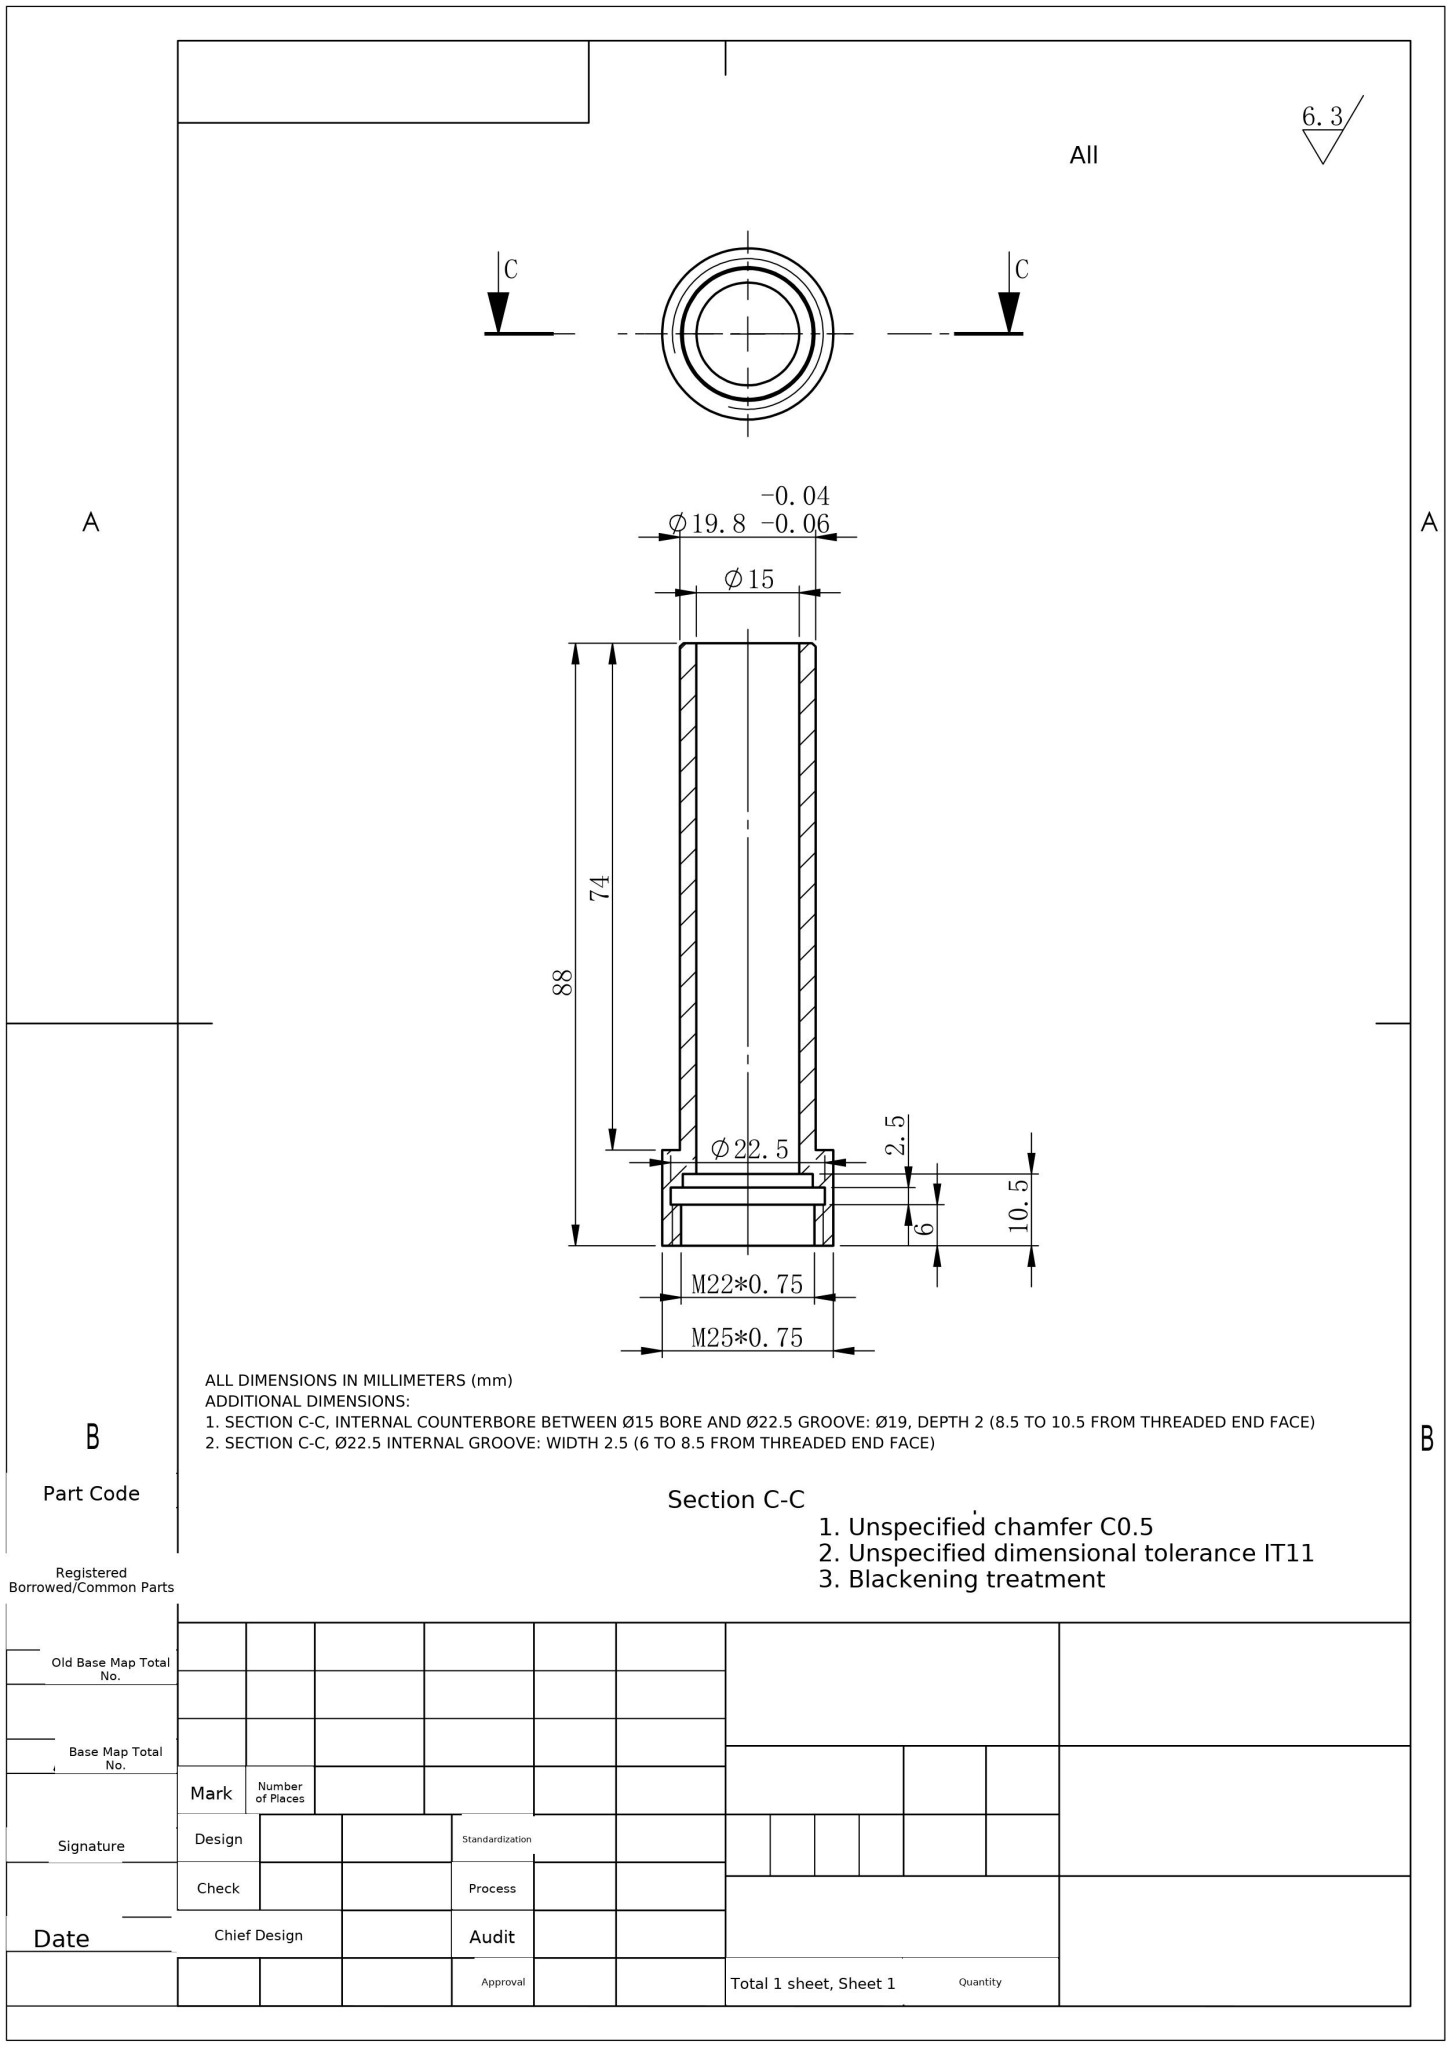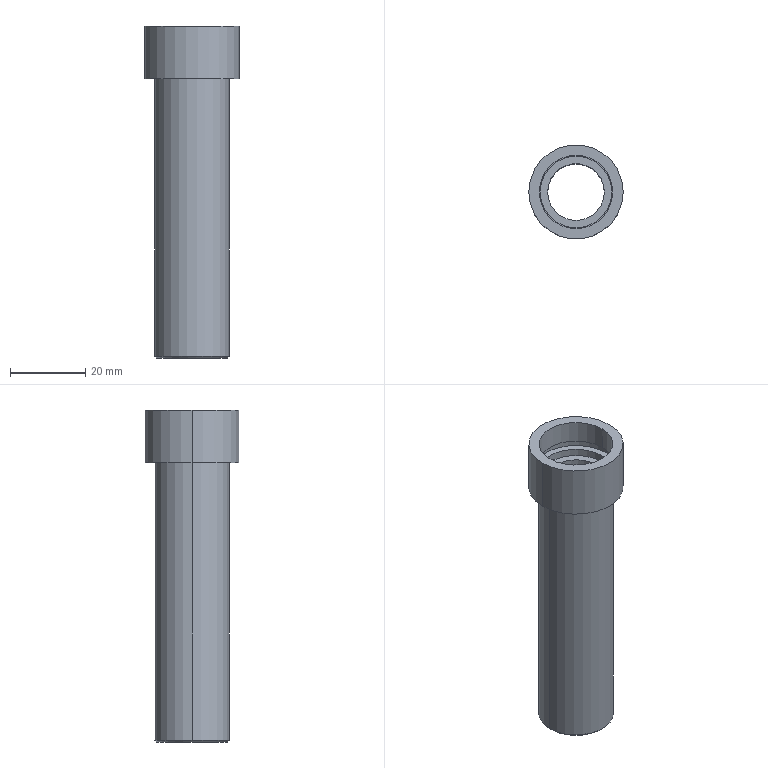Part | NX | mm | 1 solid | 20 faces | box 25 x 25 x 88 mm | volume 12601 mm3 | cylinder 12 | plane 6 | cone 2 | commonest cylinder face diameters 19 x2 25 x2 15 x2 19.8 x2 19.5 x2 22.5 x2
STEP:
#1=COLOUR_RGB('',0.5294,0.549,0.549);
#2=FILL_AREA_STYLE_COLOUR('',#1);
#3=FILL_AREA_STYLE('',(#2));
#4=SURFACE_STYLE_FILL_AREA(#3);
#5=SURFACE_SIDE_STYLE('',(#4));
#6=SURFACE_STYLE_USAGE(.BOTH.,#5);
#7=PRESENTATION_STYLE_ASSIGNMENT((#6));
#8=CARTESIAN_POINT('',(-9.4,0.,0.));
#9=VERTEX_POINT('',#8);
#10=CARTESIAN_POINT('',(9.4,0.,0.));
#11=VERTEX_POINT('',#10);
#12=CARTESIAN_POINT('',(0.,0.,0.));
#13=DIRECTION('',(0.,0.,-1.));
#14=DIRECTION('',(1.,0.,0.));
#15=AXIS2_PLACEMENT_3D('',#12,#13,#14);
#16=CIRCLE('',#15,9.4);
#17=EDGE_CURVE('',#9,#11,#16,.T.);
#18=ORIENTED_EDGE('',*,*,#17,.F.);
#19=CARTESIAN_POINT('',(-9.9,0.,0.5));
#20=VERTEX_POINT('',#19);
#21=CARTESIAN_POINT('',(-9.9,0.,0.5));
#22=DIRECTION('',(-0.7071,0.,0.7071));
#23=VECTOR('',#22,1000.);
#24=LINE('',#21,#23);
#25=EDGE_CURVE('',#9,#20,#24,.T.);
#26=ORIENTED_EDGE('',*,*,#25,.T.);
#27=CARTESIAN_POINT('',(9.9,0.,0.5));
#28=VERTEX_POINT('',#27);
#29=CARTESIAN_POINT('',(0.,0.,0.5));
#30=DIRECTION('',(0.,0.,1.));
#31=DIRECTION('',(1.,0.,0.));
#32=AXIS2_PLACEMENT_3D('',#29,#30,#31);
#33=CIRCLE('',#32,9.9);
#34=EDGE_CURVE('',#28,#20,#33,.T.);
#35=ORIENTED_EDGE('',*,*,#34,.F.);
#36=CARTESIAN_POINT('',(9.9,0.,0.5));
#37=DIRECTION('',(0.7071,0.,0.7071));
#38=VECTOR('',#37,1000.);
#39=LINE('',#36,#38);
#40=EDGE_CURVE('',#11,#28,#39,.T.);
#41=ORIENTED_EDGE('',*,*,#40,.F.);
#42=EDGE_LOOP('',(#18,#26,#35,#41));
#43=FACE_OUTER_BOUND('',#42,.T.);
#44=CARTESIAN_POINT('',(0.,0.,0.5));
#45=DIRECTION('',(0.,0.,1.));
#46=DIRECTION('',(1.,0.,0.));
#47=AXIS2_PLACEMENT_3D('',#44,#45,#46);
#48=CONICAL_SURFACE('',#47,9.9,0.7854);
#49=ADVANCED_FACE('',(#43),#48,.T.);
#50=CARTESIAN_POINT('',(-9.5,0.,77.5));
#51=VERTEX_POINT('',#50);
#52=CARTESIAN_POINT('',(9.5,0.,77.5));
#53=VERTEX_POINT('',#52);
#54=CARTESIAN_POINT('',(0.,0.,77.5));
#55=DIRECTION('',(0.,0.,1.));
#56=DIRECTION('',(1.,0.,0.));
#57=AXIS2_PLACEMENT_3D('',#54,#55,#56);
#58=CIRCLE('',#57,9.5);
#59=EDGE_CURVE('',#51,#53,#58,.T.);
#60=ORIENTED_EDGE('',*,*,#59,.F.);
#61=CARTESIAN_POINT('',(-9.5,0.,79.5));
#62=VERTEX_POINT('',#61);
#63=CARTESIAN_POINT('',(-9.5,0.,77.5));
#64=DIRECTION('',(0.,0.,1.));
#65=VECTOR('',#64,1000.);
#66=LINE('',#63,#65);
#67=EDGE_CURVE('',#51,#62,#66,.T.);
#68=ORIENTED_EDGE('',*,*,#67,.T.);
#69=CARTESIAN_POINT('',(9.5,0.,79.5));
#70=VERTEX_POINT('',#69);
#71=CARTESIAN_POINT('',(0.,0.,79.5));
#72=DIRECTION('',(0.,0.,1.));
#73=DIRECTION('',(1.,0.,0.));
#74=AXIS2_PLACEMENT_3D('',#71,#72,#73);
#75=CIRCLE('',#74,9.5);
#76=EDGE_CURVE('',#62,#70,#75,.T.);
#77=ORIENTED_EDGE('',*,*,#76,.T.);
#78=CARTESIAN_POINT('',(9.5,0.,77.5));
#79=DIRECTION('',(0.,0.,1.));
#80=VECTOR('',#79,1000.);
#81=LINE('',#78,#80);
#82=EDGE_CURVE('',#53,#70,#81,.T.);
#83=ORIENTED_EDGE('',*,*,#82,.F.);
#84=EDGE_LOOP('',(#60,#68,#77,#83));
#85=FACE_OUTER_BOUND('',#84,.T.);
#86=CARTESIAN_POINT('',(0.,0.,77.5));
#87=DIRECTION('',(0.,0.,1.));
#88=DIRECTION('',(1.,0.,0.));
#89=AXIS2_PLACEMENT_3D('',#86,#87,#88);
#90=CYLINDRICAL_SURFACE('',#89,9.5);
#91=ADVANCED_FACE('',(#85),#90,.F.);
#92=CARTESIAN_POINT('',(12.5,0.,88.));
#93=VERTEX_POINT('',#92);
#94=CARTESIAN_POINT('',(-12.5,0.,88.));
#95=VERTEX_POINT('',#94);
#96=CARTESIAN_POINT('',(0.,0.,88.));
#97=DIRECTION('',(0.,0.,1.));
#98=DIRECTION('',(1.,0.,0.));
#99=AXIS2_PLACEMENT_3D('',#96,#97,#98);
#100=CIRCLE('',#99,12.5);
#101=EDGE_CURVE('',#93,#95,#100,.T.);
#102=ORIENTED_EDGE('',*,*,#101,.F.);
#103=CARTESIAN_POINT('',(12.5,0.,74.));
#104=VERTEX_POINT('',#103);
#105=CARTESIAN_POINT('',(12.5,0.,88.));
#106=DIRECTION('',(0.,0.,-1.));
#107=VECTOR('',#106,1000.);
#108=LINE('',#105,#107);
#109=EDGE_CURVE('',#93,#104,#108,.T.);
#110=ORIENTED_EDGE('',*,*,#109,.T.);
#111=CARTESIAN_POINT('',(-12.5,0.,74.));
#112=VERTEX_POINT('',#111);
#113=CARTESIAN_POINT('',(0.,0.,74.));
#114=DIRECTION('',(0.,0.,1.));
#115=DIRECTION('',(1.,0.,0.));
#116=AXIS2_PLACEMENT_3D('',#113,#114,#115);
#117=CIRCLE('',#116,12.5);
#118=EDGE_CURVE('',#104,#112,#117,.T.);
#119=ORIENTED_EDGE('',*,*,#118,.T.);
#120=CARTESIAN_POINT('',(-12.5,0.,88.));
#121=DIRECTION('',(0.,0.,-1.));
#122=VECTOR('',#121,1000.);
#123=LINE('',#120,#122);
#124=EDGE_CURVE('',#95,#112,#123,.T.);
#125=ORIENTED_EDGE('',*,*,#124,.F.);
#126=EDGE_LOOP('',(#102,#110,#119,#125));
#127=FACE_OUTER_BOUND('',#126,.T.);
#128=CARTESIAN_POINT('',(0.,0.,88.));
#129=DIRECTION('',(0.,0.,-1.));
#130=DIRECTION('',(-1.,0.,0.));
#131=AXIS2_PLACEMENT_3D('',#128,#129,#130);
#132=CYLINDRICAL_SURFACE('',#131,12.5);
#133=ADVANCED_FACE('',(#127),#132,.T.);
#134=CARTESIAN_POINT('',(-7.5,0.,77.5));
#135=VERTEX_POINT('',#134);
#136=CARTESIAN_POINT('',(7.5,0.,77.5));
#137=VERTEX_POINT('',#136);
#138=CARTESIAN_POINT('',(0.,0.,77.5));
#139=DIRECTION('',(0.,0.,1.));
#140=DIRECTION('',(1.,0.,0.));
#141=AXIS2_PLACEMENT_3D('',#138,#139,#140);
#142=CIRCLE('',#141,7.5);
#143=EDGE_CURVE('',#135,#137,#142,.T.);
#144=ORIENTED_EDGE('',*,*,#143,.T.);
#145=CARTESIAN_POINT('',(7.5,0.,0.));
#146=VERTEX_POINT('',#145);
#147=CARTESIAN_POINT('',(7.5,0.,74.));
#148=DIRECTION('',(0.,0.,-1.));
#149=VECTOR('',#148,1000.);
#150=LINE('',#147,#149);
#151=EDGE_CURVE('',#137,#146,#150,.T.);
#152=ORIENTED_EDGE('',*,*,#151,.T.);
#153=CARTESIAN_POINT('',(-7.5,0.,0.));
#154=VERTEX_POINT('',#153);
#155=CARTESIAN_POINT('',(0.,0.,0.));
#156=DIRECTION('',(0.,0.,1.));
#157=DIRECTION('',(1.,0.,0.));
#158=AXIS2_PLACEMENT_3D('',#155,#156,#157);
#159=CIRCLE('',#158,7.5);
#160=EDGE_CURVE('',#154,#146,#159,.T.);
#161=ORIENTED_EDGE('',*,*,#160,.F.);
#162=CARTESIAN_POINT('',(-7.5,0.,74.));
#163=DIRECTION('',(0.,0.,-1.));
#164=VECTOR('',#163,1000.);
#165=LINE('',#162,#164);
#166=EDGE_CURVE('',#135,#154,#165,.T.);
#167=ORIENTED_EDGE('',*,*,#166,.F.);
#168=EDGE_LOOP('',(#144,#152,#161,#167));
#169=FACE_OUTER_BOUND('',#168,.T.);
#170=CARTESIAN_POINT('',(0.,0.,74.));
#171=DIRECTION('',(0.,0.,-1.));
#172=DIRECTION('',(-1.,0.,0.));
#173=AXIS2_PLACEMENT_3D('',#170,#171,#172);
#174=CYLINDRICAL_SURFACE('',#173,7.5);
#175=ADVANCED_FACE('',(#169),#174,.F.);
#176=CARTESIAN_POINT('',(9.9,0.,74.));
#177=VERTEX_POINT('',#176);
#178=CARTESIAN_POINT('',(-9.9,0.,74.));
#179=VERTEX_POINT('',#178);
#180=CARTESIAN_POINT('',(0.,0.,74.));
#181=DIRECTION('',(0.,0.,1.));
#182=DIRECTION('',(1.,0.,0.));
#183=AXIS2_PLACEMENT_3D('',#180,#181,#182);
#184=CIRCLE('',#183,9.9);
#185=EDGE_CURVE('',#177,#179,#184,.T.);
#186=ORIENTED_EDGE('',*,*,#185,.F.);
#187=CARTESIAN_POINT('',(9.9,0.,74.));
#188=DIRECTION('',(0.,0.,-1.));
#189=VECTOR('',#188,1000.);
#190=LINE('',#187,#189);
#191=EDGE_CURVE('',#177,#28,#190,.T.);
#192=ORIENTED_EDGE('',*,*,#191,.T.);
#193=ORIENTED_EDGE('',*,*,#34,.T.);
#194=CARTESIAN_POINT('',(-9.9,0.,74.));
#195=DIRECTION('',(0.,0.,-1.));
#196=VECTOR('',#195,1000.);
#197=LINE('',#194,#196);
#198=EDGE_CURVE('',#179,#20,#197,.T.);
#199=ORIENTED_EDGE('',*,*,#198,.F.);
#200=EDGE_LOOP('',(#186,#192,#193,#199));
#201=FACE_OUTER_BOUND('',#200,.T.);
#202=CARTESIAN_POINT('',(0.,0.,74.));
#203=DIRECTION('',(0.,0.,-1.));
#204=DIRECTION('',(-1.,0.,0.));
#205=AXIS2_PLACEMENT_3D('',#202,#203,#204);
#206=CYLINDRICAL_SURFACE('',#205,9.9);
#207=ADVANCED_FACE('',(#201),#206,.T.);
#208=CARTESIAN_POINT('',(-9.75,0.,82.));
#209=VERTEX_POINT('',#208);
#210=CARTESIAN_POINT('',(9.75,0.,82.));
#211=VERTEX_POINT('',#210);
#212=CARTESIAN_POINT('',(0.,0.,82.));
#213=DIRECTION('',(0.,0.,1.));
#214=DIRECTION('',(1.,0.,0.));
#215=AXIS2_PLACEMENT_3D('',#212,#213,#214);
#216=CIRCLE('',#215,9.75);
#217=EDGE_CURVE('',#209,#211,#216,.T.);
#218=ORIENTED_EDGE('',*,*,#217,.F.);
#219=CARTESIAN_POINT('',(-9.75,0.,88.));
#220=VERTEX_POINT('',#219);
#221=CARTESIAN_POINT('',(-9.75,0.,88.));
#222=DIRECTION('',(0.,0.,1.));
#223=VECTOR('',#222,1000.);
#224=LINE('',#221,#223);
#225=EDGE_CURVE('',#209,#220,#224,.T.);
#226=ORIENTED_EDGE('',*,*,#225,.T.);
#227=CARTESIAN_POINT('',(9.75,0.,88.));
#228=VERTEX_POINT('',#227);
#229=CARTESIAN_POINT('',(0.,0.,88.));
#230=DIRECTION('',(0.,0.,1.));
#231=DIRECTION('',(1.,0.,0.));
#232=AXIS2_PLACEMENT_3D('',#229,#230,#231);
#233=CIRCLE('',#232,9.75);
#234=EDGE_CURVE('',#220,#228,#233,.T.);
#235=ORIENTED_EDGE('',*,*,#234,.T.);
#236=CARTESIAN_POINT('',(9.75,0.,88.));
#237=DIRECTION('',(0.,0.,1.));
#238=VECTOR('',#237,1000.);
#239=LINE('',#236,#238);
#240=EDGE_CURVE('',#211,#228,#239,.T.);
#241=ORIENTED_EDGE('',*,*,#240,.F.);
#242=EDGE_LOOP('',(#218,#226,#235,#241));
#243=FACE_OUTER_BOUND('',#242,.T.);
#244=CARTESIAN_POINT('',(0.,0.,88.));
#245=DIRECTION('',(0.,0.,1.));
#246=DIRECTION('',(1.,0.,0.));
#247=AXIS2_PLACEMENT_3D('',#244,#245,#246);
#248=CYLINDRICAL_SURFACE('',#247,9.75);
#249=ADVANCED_FACE('',(#243),#248,.F.);
#250=CARTESIAN_POINT('',(-11.25,0.,79.5));
#251=VERTEX_POINT('',#250);
#252=CARTESIAN_POINT('',(11.25,0.,79.5));
#253=VERTEX_POINT('',#252);
#254=CARTESIAN_POINT('',(0.,0.,79.5));
#255=DIRECTION('',(0.,0.,1.));
#256=DIRECTION('',(1.,0.,0.));
#257=AXIS2_PLACEMENT_3D('',#254,#255,#256);
#258=CIRCLE('',#257,11.25);
#259=EDGE_CURVE('',#251,#253,#258,.T.);
#260=ORIENTED_EDGE('',*,*,#259,.F.);
#261=CARTESIAN_POINT('',(-11.25,0.,82.));
#262=VERTEX_POINT('',#261);
#263=CARTESIAN_POINT('',(-11.25,0.,79.5));
#264=DIRECTION('',(0.,0.,1.));
#265=VECTOR('',#264,1000.);
#266=LINE('',#263,#265);
#267=EDGE_CURVE('',#251,#262,#266,.T.);
#268=ORIENTED_EDGE('',*,*,#267,.T.);
#269=CARTESIAN_POINT('',(11.25,0.,82.));
#270=VERTEX_POINT('',#269);
#271=CARTESIAN_POINT('',(0.,0.,82.));
#272=DIRECTION('',(0.,0.,1.));
#273=DIRECTION('',(1.,0.,0.));
#274=AXIS2_PLACEMENT_3D('',#271,#272,#273);
#275=CIRCLE('',#274,11.25);
#276=EDGE_CURVE('',#262,#270,#275,.T.);
#277=ORIENTED_EDGE('',*,*,#276,.T.);
#278=CARTESIAN_POINT('',(11.25,0.,79.5));
#279=DIRECTION('',(0.,0.,1.));
#280=VECTOR('',#279,1000.);
#281=LINE('',#278,#280);
#282=EDGE_CURVE('',#253,#270,#281,.T.);
#283=ORIENTED_EDGE('',*,*,#282,.F.);
#284=EDGE_LOOP('',(#260,#268,#277,#283));
#285=FACE_OUTER_BOUND('',#284,.T.);
#286=CARTESIAN_POINT('',(0.,0.,79.5));
#287=DIRECTION('',(0.,0.,1.));
#288=DIRECTION('',(1.,0.,0.));
#289=AXIS2_PLACEMENT_3D('',#286,#287,#288);
#290=CYLINDRICAL_SURFACE('',#289,11.25);
#291=ADVANCED_FACE('',(#285),#290,.F.);
#292=ORIENTED_EDGE('',*,*,#267,.F.);
#293=CARTESIAN_POINT('',(0.,0.,79.5));
#294=DIRECTION('',(0.,0.,1.));
#295=DIRECTION('',(1.,0.,0.));
#296=AXIS2_PLACEMENT_3D('',#293,#294,#295);
#297=CIRCLE('',#296,11.25);
#298=EDGE_CURVE('',#253,#251,#297,.T.);
#299=ORIENTED_EDGE('',*,*,#298,.F.);
#300=ORIENTED_EDGE('',*,*,#282,.T.);
#301=CARTESIAN_POINT('',(0.,0.,82.));
#302=DIRECTION('',(0.,0.,1.));
#303=DIRECTION('',(1.,0.,0.));
#304=AXIS2_PLACEMENT_3D('',#301,#302,#303);
#305=CIRCLE('',#304,11.25);
#306=EDGE_CURVE('',#270,#262,#305,.T.);
#307=ORIENTED_EDGE('',*,*,#306,.T.);
#308=EDGE_LOOP('',(#292,#299,#300,#307));
#309=FACE_OUTER_BOUND('',#308,.T.);
#310=CARTESIAN_POINT('',(0.,0.,79.5));
#311=DIRECTION('',(0.,0.,1.));
#312=DIRECTION('',(1.,0.,0.));
#313=AXIS2_PLACEMENT_3D('',#310,#311,#312);
#314=CYLINDRICAL_SURFACE('',#313,11.25);
#315=ADVANCED_FACE('',(#309),#314,.F.);
#316=CARTESIAN_POINT('',(0.,0.,79.5));
#317=DIRECTION('',(0.,0.,1.));
#318=DIRECTION('',(1.,0.,0.));
#319=AXIS2_PLACEMENT_3D('',#316,#317,#318);
#320=CIRCLE('',#319,9.5);
#321=EDGE_CURVE('',#70,#62,#320,.T.);
#322=ORIENTED_EDGE('',*,*,#321,.F.);
#323=ORIENTED_EDGE('',*,*,#76,.F.);
#324=EDGE_LOOP('',(#322,#323));
#325=FACE_BOUND('',#324,.T.);
#326=ORIENTED_EDGE('',*,*,#298,.T.);
#327=ORIENTED_EDGE('',*,*,#259,.T.);
#328=EDGE_LOOP('',(#326,#327));
#329=FACE_OUTER_BOUND('',#328,.T.);
#330=CARTESIAN_POINT('',(0.,0.,79.5));
#331=DIRECTION('',(0.,0.,1.));
#332=DIRECTION('',(1.,0.,0.));
#333=AXIS2_PLACEMENT_3D('',#330,#331,#332);
#334=PLANE('',#333);
#335=ADVANCED_FACE('',(#325,#329),#334,.T.);
#336=CARTESIAN_POINT('',(0.,0.,82.));
#337=DIRECTION('',(0.,0.,1.));
#338=DIRECTION('',(1.,0.,0.));
#339=AXIS2_PLACEMENT_3D('',#336,#337,#338);
#340=CIRCLE('',#339,9.75);
#341=EDGE_CURVE('',#211,#209,#340,.T.);
#342=ORIENTED_EDGE('',*,*,#341,.T.);
#343=ORIENTED_EDGE('',*,*,#217,.T.);
#344=EDGE_LOOP('',(#342,#343));
#345=FACE_BOUND('',#344,.T.);
#346=ORIENTED_EDGE('',*,*,#306,.F.);
#347=ORIENTED_EDGE('',*,*,#276,.F.);
#348=EDGE_LOOP('',(#346,#347));
#349=FACE_OUTER_BOUND('',#348,.T.);
#350=CARTESIAN_POINT('',(0.,0.,82.));
#351=DIRECTION('',(0.,0.,1.));
#352=DIRECTION('',(1.,0.,0.));
#353=AXIS2_PLACEMENT_3D('',#350,#351,#352);
#354=PLANE('',#353);
#355=ADVANCED_FACE('',(#345,#349),#354,.F.);
#356=ORIENTED_EDGE('',*,*,#225,.F.);
#357=ORIENTED_EDGE('',*,*,#341,.F.);
#358=ORIENTED_EDGE('',*,*,#240,.T.);
#359=CARTESIAN_POINT('',(0.,0.,88.));
#360=DIRECTION('',(0.,0.,1.));
#361=DIRECTION('',(1.,0.,0.));
#362=AXIS2_PLACEMENT_3D('',#359,#360,#361);
#363=CIRCLE('',#362,9.75);
#364=EDGE_CURVE('',#228,#220,#363,.T.);
#365=ORIENTED_EDGE('',*,*,#364,.T.);
#366=EDGE_LOOP('',(#356,#357,#358,#365));
#367=FACE_OUTER_BOUND('',#366,.T.);
#368=CARTESIAN_POINT('',(0.,0.,88.));
#369=DIRECTION('',(0.,0.,1.));
#370=DIRECTION('',(1.,0.,0.));
#371=AXIS2_PLACEMENT_3D('',#368,#369,#370);
#372=CYLINDRICAL_SURFACE('',#371,9.75);
#373=ADVANCED_FACE('',(#367),#372,.F.);
#374=CARTESIAN_POINT('',(0.,0.,0.));
#375=DIRECTION('',(0.,0.,-1.));
#376=DIRECTION('',(1.,0.,0.));
#377=AXIS2_PLACEMENT_3D('',#374,#375,#376);
#378=CIRCLE('',#377,9.4);
#379=EDGE_CURVE('',#11,#9,#378,.T.);
#380=ORIENTED_EDGE('',*,*,#379,.T.);
#381=ORIENTED_EDGE('',*,*,#17,.T.);
#382=EDGE_LOOP('',(#380,#381));
#383=FACE_OUTER_BOUND('',#382,.T.);
#384=ORIENTED_EDGE('',*,*,#160,.T.);
#385=CARTESIAN_POINT('',(0.,0.,0.));
#386=DIRECTION('',(0.,0.,1.));
#387=DIRECTION('',(1.,0.,0.));
#388=AXIS2_PLACEMENT_3D('',#385,#386,#387);
#389=CIRCLE('',#388,7.5);
#390=EDGE_CURVE('',#146,#154,#389,.T.);
#391=ORIENTED_EDGE('',*,*,#390,.T.);
#392=EDGE_LOOP('',(#384,#391));
#393=FACE_BOUND('',#392,.T.);
#394=CARTESIAN_POINT('',(0.,0.,0.));
#395=DIRECTION('',(0.,0.,1.));
#396=DIRECTION('',(1.,0.,0.));
#397=AXIS2_PLACEMENT_3D('',#394,#395,#396);
#398=PLANE('',#397);
#399=ADVANCED_FACE('',(#383,#393),#398,.F.);
#400=ORIENTED_EDGE('',*,*,#191,.F.);
#401=CARTESIAN_POINT('',(0.,0.,74.));
#402=DIRECTION('',(0.,0.,1.));
#403=DIRECTION('',(1.,0.,0.));
#404=AXIS2_PLACEMENT_3D('',#401,#402,#403);
#405=CIRCLE('',#404,9.9);
#406=EDGE_CURVE('',#179,#177,#405,.T.);
#407=ORIENTED_EDGE('',*,*,#406,.F.);
#408=ORIENTED_EDGE('',*,*,#198,.T.);
#409=CARTESIAN_POINT('',(0.,0.,0.5));
#410=DIRECTION('',(0.,0.,1.));
#411=DIRECTION('',(1.,0.,0.));
#412=AXIS2_PLACEMENT_3D('',#409,#410,#411);
#413=CIRCLE('',#412,9.9);
#414=EDGE_CURVE('',#20,#28,#413,.T.);
#415=ORIENTED_EDGE('',*,*,#414,.T.);
#416=EDGE_LOOP('',(#400,#407,#408,#415));
#417=FACE_OUTER_BOUND('',#416,.T.);
#418=CARTESIAN_POINT('',(0.,0.,74.));
#419=DIRECTION('',(0.,0.,-1.));
#420=DIRECTION('',(-1.,0.,0.));
#421=AXIS2_PLACEMENT_3D('',#418,#419,#420);
#422=CYLINDRICAL_SURFACE('',#421,9.9);
#423=ADVANCED_FACE('',(#417),#422,.T.);
#424=ORIENTED_EDGE('',*,*,#151,.F.);
#425=CARTESIAN_POINT('',(0.,0.,77.5));
#426=DIRECTION('',(0.,0.,1.));
#427=DIRECTION('',(1.,0.,0.));
#428=AXIS2_PLACEMENT_3D('',#425,#426,#427);
#429=CIRCLE('',#428,7.5);
#430=EDGE_CURVE('',#137,#135,#429,.T.);
#431=ORIENTED_EDGE('',*,*,#430,.T.);
#432=ORIENTED_EDGE('',*,*,#166,.T.);
#433=ORIENTED_EDGE('',*,*,#390,.F.);
#434=EDGE_LOOP('',(#424,#431,#432,#433));
#435=FACE_OUTER_BOUND('',#434,.T.);
#436=CARTESIAN_POINT('',(0.,0.,74.));
#437=DIRECTION('',(0.,0.,-1.));
#438=DIRECTION('',(-1.,0.,0.));
#439=AXIS2_PLACEMENT_3D('',#436,#437,#438);
#440=CYLINDRICAL_SURFACE('',#439,7.5);
#441=ADVANCED_FACE('',(#435),#440,.F.);
#442=CARTESIAN_POINT('',(0.,0.,74.));
#443=DIRECTION('',(0.,0.,1.));
#444=DIRECTION('',(1.,0.,0.));
#445=AXIS2_PLACEMENT_3D('',#442,#443,#444);
#446=CIRCLE('',#445,12.5);
#447=EDGE_CURVE('',#112,#104,#446,.T.);
#448=ORIENTED_EDGE('',*,*,#447,.F.);
#449=ORIENTED_EDGE('',*,*,#118,.F.);
#450=EDGE_LOOP('',(#448,#449));
#451=FACE_OUTER_BOUND('',#450,.T.);
#452=ORIENTED_EDGE('',*,*,#406,.T.);
#453=ORIENTED_EDGE('',*,*,#185,.T.);
#454=EDGE_LOOP('',(#452,#453));
#455=FACE_BOUND('',#454,.T.);
#456=CARTESIAN_POINT('',(0.,0.,74.));
#457=DIRECTION('',(0.,0.,1.));
#458=DIRECTION('',(1.,0.,0.));
#459=AXIS2_PLACEMENT_3D('',#456,#457,#458);
#460=PLANE('',#459);
#461=ADVANCED_FACE('',(#451,#455),#460,.F.);
#462=ORIENTED_EDGE('',*,*,#109,.F.);
#463=CARTESIAN_POINT('',(0.,0.,88.));
#464=DIRECTION('',(0.,0.,1.));
#465=DIRECTION('',(1.,0.,0.));
#466=AXIS2_PLACEMENT_3D('',#463,#464,#465);
#467=CIRCLE('',#466,12.5);
#468=EDGE_CURVE('',#95,#93,#467,.T.);
#469=ORIENTED_EDGE('',*,*,#468,.F.);
#470=ORIENTED_EDGE('',*,*,#124,.T.);
#471=ORIENTED_EDGE('',*,*,#447,.T.);
#472=EDGE_LOOP('',(#462,#469,#470,#471));
#473=FACE_OUTER_BOUND('',#472,.T.);
#474=CARTESIAN_POINT('',(0.,0.,88.));
#475=DIRECTION('',(0.,0.,-1.));
#476=DIRECTION('',(-1.,0.,0.));
#477=AXIS2_PLACEMENT_3D('',#474,#475,#476);
#478=CYLINDRICAL_SURFACE('',#477,12.5);
#479=ADVANCED_FACE('',(#473),#478,.T.);
#480=ORIENTED_EDGE('',*,*,#364,.F.);
#481=ORIENTED_EDGE('',*,*,#234,.F.);
#482=EDGE_LOOP('',(#480,#481));
#483=FACE_BOUND('',#482,.T.);
#484=ORIENTED_EDGE('',*,*,#468,.T.);
#485=ORIENTED_EDGE('',*,*,#101,.T.);
#486=EDGE_LOOP('',(#484,#485));
#487=FACE_OUTER_BOUND('',#486,.T.);
#488=CARTESIAN_POINT('',(0.,0.,88.));
#489=DIRECTION('',(0.,0.,1.));
#490=DIRECTION('',(1.,0.,0.));
#491=AXIS2_PLACEMENT_3D('',#488,#489,#490);
#492=PLANE('',#491);
#493=ADVANCED_FACE('',(#483,#487),#492,.T.);
#494=ORIENTED_EDGE('',*,*,#67,.F.);
#495=CARTESIAN_POINT('',(0.,0.,77.5));
#496=DIRECTION('',(0.,0.,1.));
#497=DIRECTION('',(1.,0.,0.));
#498=AXIS2_PLACEMENT_3D('',#495,#496,#497);
#499=CIRCLE('',#498,9.5);
#500=EDGE_CURVE('',#53,#51,#499,.T.);
#501=ORIENTED_EDGE('',*,*,#500,.F.);
#502=ORIENTED_EDGE('',*,*,#82,.T.);
#503=ORIENTED_EDGE('',*,*,#321,.T.);
#504=EDGE_LOOP('',(#494,#501,#502,#503));
#505=FACE_OUTER_BOUND('',#504,.T.);
#506=CARTESIAN_POINT('',(0.,0.,77.5));
#507=DIRECTION('',(0.,0.,1.));
#508=DIRECTION('',(1.,0.,0.));
#509=AXIS2_PLACEMENT_3D('',#506,#507,#508);
#510=CYLINDRICAL_SURFACE('',#509,9.5);
#511=ADVANCED_FACE('',(#505),#510,.F.);
#512=ORIENTED_EDGE('',*,*,#143,.F.);
#513=ORIENTED_EDGE('',*,*,#430,.F.);
#514=EDGE_LOOP('',(#512,#513));
#515=FACE_BOUND('',#514,.T.);
#516=ORIENTED_EDGE('',*,*,#500,.T.);
#517=ORIENTED_EDGE('',*,*,#59,.T.);
#518=EDGE_LOOP('',(#516,#517));
#519=FACE_OUTER_BOUND('',#518,.T.);
#520=CARTESIAN_POINT('',(0.,0.,77.5));
#521=DIRECTION('',(0.,0.,1.));
#522=DIRECTION('',(1.,0.,0.));
#523=AXIS2_PLACEMENT_3D('',#520,#521,#522);
#524=PLANE('',#523);
#525=ADVANCED_FACE('',(#515,#519),#524,.T.);
#526=ORIENTED_EDGE('',*,*,#25,.F.);
#527=ORIENTED_EDGE('',*,*,#379,.F.);
#528=ORIENTED_EDGE('',*,*,#40,.T.);
#529=ORIENTED_EDGE('',*,*,#414,.F.);
#530=EDGE_LOOP('',(#526,#527,#528,#529));
#531=FACE_OUTER_BOUND('',#530,.T.);
#532=CARTESIAN_POINT('',(0.,0.,0.5));
#533=DIRECTION('',(0.,0.,1.));
#534=DIRECTION('',(1.,0.,0.));
#535=AXIS2_PLACEMENT_3D('',#532,#533,#534);
#536=CONICAL_SURFACE('',#535,9.9,0.7854);
#537=ADVANCED_FACE('',(#531),#536,.T.);
#538=CLOSED_SHELL('',(#49,#91,#133,#175,#207,#249,#291,#315,#335,#355,#373,#399,#423,#441,#461,#479,#493,#511,#525,#537));
#539=MANIFOLD_SOLID_BREP('',#538);
#540=CARTESIAN_POINT('',(0.,0.,0.));
#541=DIRECTION('',(0.,0.,1.));
#542=DIRECTION('',(1.,0.,0.));
#543=AXIS2_PLACEMENT_3D('',#540,#541,#542);
#544=(LENGTH_UNIT()NAMED_UNIT(*)SI_UNIT(.MILLI.,.METRE.));
#545=UNCERTAINTY_MEASURE_WITH_UNIT(LENGTH_MEASURE(0.00001),#544,'','');
#546=(NAMED_UNIT(*)PLANE_ANGLE_UNIT()SI_UNIT($,.RADIAN.));
#547=(NAMED_UNIT(*)SI_UNIT($,.STERADIAN.)SOLID_ANGLE_UNIT());
#548=(GEOMETRIC_REPRESENTATION_CONTEXT(3)GLOBAL_UNCERTAINTY_ASSIGNED_CONTEXT((#545))GLOBAL_UNIT_ASSIGNED_CONTEXT((#544,#546,#547))REPRESENTATION_CONTEXT('',''));
#549=ADVANCED_BREP_SHAPE_REPRESENTATION('',(#539,#543),#548);
#550=STYLED_ITEM('',(#7),#549);
#551=PRESENTATION_LAYER_ASSIGNMENT('','',(#550));
#552=COLOUR_RGB('',0.5294,0.549,0.549);
#553=FILL_AREA_STYLE_COLOUR('',#552);
#554=FILL_AREA_STYLE('',(#553));
#555=SURFACE_STYLE_FILL_AREA(#554);
#556=SURFACE_SIDE_STYLE('',(#555));
#557=SURFACE_STYLE_USAGE(.BOTH.,#556);
#558=PRESENTATION_STYLE_ASSIGNMENT((#557));
#559=STYLED_ITEM('',(#558),#133);
#560=PRESENTATION_LAYER_ASSIGNMENT('','',(#559));
#561=COLOUR_RGB('',0.5294,0.549,0.549);
#562=FILL_AREA_STYLE_COLOUR('',#561);
#563=FILL_AREA_STYLE('',(#562));
#564=SURFACE_STYLE_FILL_AREA(#563);
#565=SURFACE_SIDE_STYLE('',(#564));
#566=SURFACE_STYLE_USAGE(.BOTH.,#565);
#567=PRESENTATION_STYLE_ASSIGNMENT((#566));
#568=STYLED_ITEM('',(#567),#539);
#569=PRESENTATION_LAYER_ASSIGNMENT('','',(#568));
#570=COLOUR_RGB('',0.5294,0.549,0.549);
#571=FILL_AREA_STYLE_COLOUR('',#570);
#572=FILL_AREA_STYLE('',(#571));
#573=SURFACE_STYLE_FILL_AREA(#572);
#574=SURFACE_SIDE_STYLE('',(#573));
#575=SURFACE_STYLE_USAGE(.BOTH.,#574);
#576=PRESENTATION_STYLE_ASSIGNMENT((#575));
#577=STYLED_ITEM('',(#576),#373);
#578=(LENGTH_UNIT()NAMED_UNIT(*)SI_UNIT(.MILLI.,.METRE.));
#579=UNCERTAINTY_MEASURE_WITH_UNIT(LENGTH_MEASURE(0.00001),#578,'','');
#580=(NAMED_UNIT(*)PLANE_ANGLE_UNIT()SI_UNIT($,.RADIAN.));
#581=(NAMED_UNIT(*)SI_UNIT($,.STERADIAN.)SOLID_ANGLE_UNIT());
#582=(GEOMETRIC_REPRESENTATION_CONTEXT(3)GLOBAL_UNCERTAINTY_ASSIGNED_CONTEXT((#579))GLOBAL_UNIT_ASSIGNED_CONTEXT((#578,#580,#581))REPRESENTATION_CONTEXT('',''));
#583=MECHANICAL_DESIGN_GEOMETRIC_PRESENTATION_REPRESENTATION('',(#577),#582);
#584=COLOUR_RGB('',0.5294,0.549,0.549);
#585=FILL_AREA_STYLE_COLOUR('',#584);
#586=FILL_AREA_STYLE('',(#585));
#587=SURFACE_STYLE_FILL_AREA(#586);
#588=SURFACE_SIDE_STYLE('',(#587));
#589=SURFACE_STYLE_USAGE(.BOTH.,#588);
#590=PRESENTATION_STYLE_ASSIGNMENT((#589));
#591=STYLED_ITEM('',(#590),#479);
#592=(LENGTH_UNIT()NAMED_UNIT(*)SI_UNIT(.MILLI.,.METRE.));
#593=UNCERTAINTY_MEASURE_WITH_UNIT(LENGTH_MEASURE(0.00001),#592,'','');
#594=(NAMED_UNIT(*)PLANE_ANGLE_UNIT()SI_UNIT($,.RADIAN.));
#595=(NAMED_UNIT(*)SI_UNIT($,.STERADIAN.)SOLID_ANGLE_UNIT());
#596=(GEOMETRIC_REPRESENTATION_CONTEXT(3)GLOBAL_UNCERTAINTY_ASSIGNED_CONTEXT((#593))GLOBAL_UNIT_ASSIGNED_CONTEXT((#592,#594,#595))REPRESENTATION_CONTEXT('',''));
#597=MECHANICAL_DESIGN_GEOMETRIC_PRESENTATION_REPRESENTATION('',(#591),#596);
#598=COLOUR_RGB('',0.5294,0.549,0.549);
#599=FILL_AREA_STYLE_COLOUR('',#598);
#600=FILL_AREA_STYLE('',(#599));
#601=SURFACE_STYLE_FILL_AREA(#600);
#602=SURFACE_SIDE_STYLE('',(#601));
#603=SURFACE_STYLE_USAGE(.BOTH.,#602);
#604=PRESENTATION_STYLE_ASSIGNMENT((#603));
#605=STYLED_ITEM('',(#604),#249);
#606=(LENGTH_UNIT()NAMED_UNIT(*)SI_UNIT(.MILLI.,.METRE.));
#607=UNCERTAINTY_MEASURE_WITH_UNIT(LENGTH_MEASURE(0.00001),#606,'','');
#608=(NAMED_UNIT(*)PLANE_ANGLE_UNIT()SI_UNIT($,.RADIAN.));
#609=(NAMED_UNIT(*)SI_UNIT($,.STERADIAN.)SOLID_ANGLE_UNIT());
#610=(GEOMETRIC_REPRESENTATION_CONTEXT(3)GLOBAL_UNCERTAINTY_ASSIGNED_CONTEXT((#607))GLOBAL_UNIT_ASSIGNED_CONTEXT((#606,#608,#609))REPRESENTATION_CONTEXT('',''));
#611=MECHANICAL_DESIGN_GEOMETRIC_PRESENTATION_REPRESENTATION('',(#605),#610);
#612=(LENGTH_UNIT()NAMED_UNIT(*)SI_UNIT(.MILLI.,.METRE.));
#613=UNCERTAINTY_MEASURE_WITH_UNIT(LENGTH_MEASURE(0.00001),#612,'','');
#614=(NAMED_UNIT(*)PLANE_ANGLE_UNIT()SI_UNIT($,.RADIAN.));
#615=(NAMED_UNIT(*)SI_UNIT($,.STERADIAN.)SOLID_ANGLE_UNIT());
#616=(GEOMETRIC_REPRESENTATION_CONTEXT(3)GLOBAL_UNCERTAINTY_ASSIGNED_CONTEXT((#613))GLOBAL_UNIT_ASSIGNED_CONTEXT((#612,#614,#615))REPRESENTATION_CONTEXT('',''));
#617=MECHANICAL_DESIGN_GEOMETRIC_PRESENTATION_REPRESENTATION('',(#550),#616);
#618=(LENGTH_UNIT()NAMED_UNIT(*)SI_UNIT(.MILLI.,.METRE.));
#619=UNCERTAINTY_MEASURE_WITH_UNIT(LENGTH_MEASURE(0.00001),#618,'','');
#620=(NAMED_UNIT(*)PLANE_ANGLE_UNIT()SI_UNIT($,.RADIAN.));
#621=(NAMED_UNIT(*)SI_UNIT($,.STERADIAN.)SOLID_ANGLE_UNIT());
#622=(GEOMETRIC_REPRESENTATION_CONTEXT(3)GLOBAL_UNCERTAINTY_ASSIGNED_CONTEXT((#619))GLOBAL_UNIT_ASSIGNED_CONTEXT((#618,#620,#621))REPRESENTATION_CONTEXT('',''));
#623=MECHANICAL_DESIGN_GEOMETRIC_PRESENTATION_REPRESENTATION('',(#559),#622);
#624=PRESENTATION_LAYER_ASSIGNMENT('','',(#577));
#625=(LENGTH_UNIT()NAMED_UNIT(*)SI_UNIT(.MILLI.,.METRE.));
#626=UNCERTAINTY_MEASURE_WITH_UNIT(LENGTH_MEASURE(0.00001),#625,'','');
#627=(NAMED_UNIT(*)PLANE_ANGLE_UNIT()SI_UNIT($,.RADIAN.));
#628=(NAMED_UNIT(*)SI_UNIT($,.STERADIAN.)SOLID_ANGLE_UNIT());
#629=(GEOMETRIC_REPRESENTATION_CONTEXT(3)GLOBAL_UNCERTAINTY_ASSIGNED_CONTEXT((#626))GLOBAL_UNIT_ASSIGNED_CONTEXT((#625,#627,#628))REPRESENTATION_CONTEXT('',''));
#630=MECHANICAL_DESIGN_GEOMETRIC_PRESENTATION_REPRESENTATION('',(#568),#629);
#631=PRESENTATION_LAYER_ASSIGNMENT('','',(#591));
#632=PRESENTATION_LAYER_ASSIGNMENT('','',(#605));